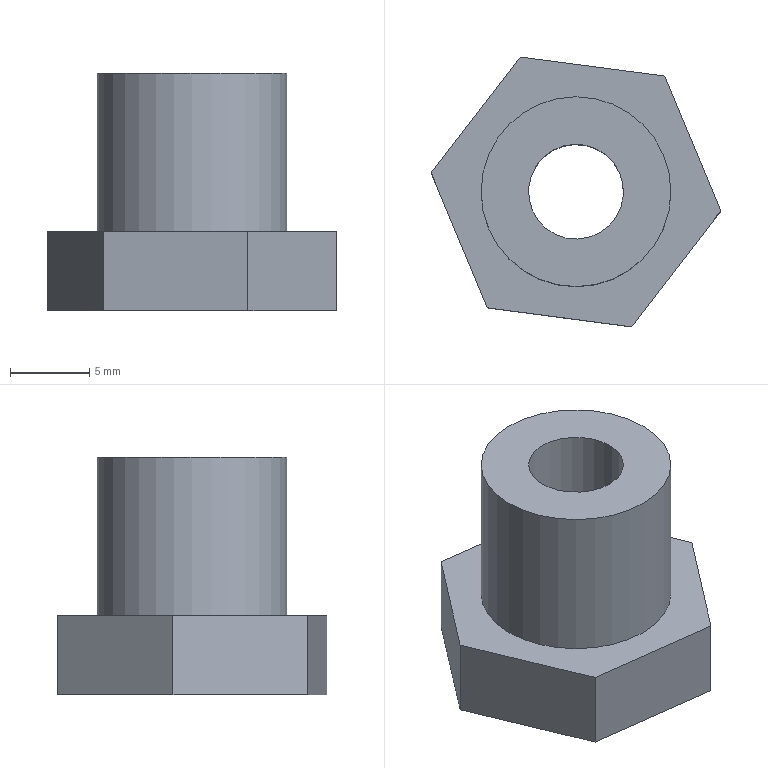Component | NX | 08__27_2 | 1 solid | 11 faces | box 18.32 x 17.07 x 15 mm | volume 1815 mm3 | plane 9 | cylinder 2 | commonest cylinder face diameters 6 x1 12 x1
STEP:
#1=CARTESIAN_POINT('',(0.,0.,0.));
#2=DIRECTION('',(0.,0.,1.));
#3=DIRECTION('',(1.,0.,0.));
#4=AXIS2_PLACEMENT_3D('',#1,#2,#3);
#5=CARTESIAN_POINT('',(110.402,102.277,172.432));
#6=VERTEX_POINT('',#5);
#7=CARTESIAN_POINT('',(106.863,110.81,172.432));
#8=VERTEX_POINT('',#7);
#9=CARTESIAN_POINT('',(110.402,102.277,172.432));
#10=DIRECTION('',(-0.383,0.9237,0.));
#11=VECTOR('',#10,1.);
#12=LINE('',#9,#11);
#13=CARTESIAN_POINT('',(110.402,102.277,167.432));
#14=DIRECTION('',(0.9237,0.383,0.));
#15=DIRECTION('',(0.383,-0.9237,0.));
#16=AXIS2_PLACEMENT_3D('',#13,#14,#15);
#17=PLANE('',#16);
#18=CARTESIAN_POINT('',(0.,-5.));
#19=DIRECTION('',(-1.,0.));
#20=VECTOR('',#19,1.);
#21=LINE('',#18,#20);
#22=(GEOMETRIC_REPRESENTATION_CONTEXT(2)PARAMETRIC_REPRESENTATION_CONTEXT()REPRESENTATION_CONTEXT('',''));
#23=DEFINITIONAL_REPRESENTATION('',(#21),#22);
#24=PCURVE('',#17,#23);
#25=CARTESIAN_POINT('',(116.022,109.608,172.432));
#26=DIRECTION('',(0.,0.,-1.));
#27=DIRECTION('',(0.9237,0.383,0.));
#28=AXIS2_PLACEMENT_3D('',#25,#26,#27);
#29=PLANE('',#28);
#30=CARTESIAN_POINT('',(-8.,4.619));
#31=DIRECTION('',(-0.,-1.));
#32=VECTOR('',#31,1.);
#33=LINE('',#30,#32);
#34=(GEOMETRIC_REPRESENTATION_CONTEXT(2)PARAMETRIC_REPRESENTATION_CONTEXT()REPRESENTATION_CONTEXT('',''));
#35=DEFINITIONAL_REPRESENTATION('',(#33),#34);
#36=PCURVE('',#29,#35);
#37=SURFACE_CURVE('',#12,(#24,#36),.PCURVE_S1.);
#38=EDGE_CURVE('',#6,#8,#37,.T.);
#39=ORIENTED_EDGE('',*,*,#38,.T.);
#40=CARTESIAN_POINT('',(106.863,110.81,167.432));
#41=VERTEX_POINT('',#40);
#42=CARTESIAN_POINT('',(106.863,110.81,167.432));
#43=DIRECTION('',(0.,0.,1.));
#44=VECTOR('',#43,1.);
#45=LINE('',#42,#44);
#46=CARTESIAN_POINT('',(-9.238,0.));
#47=DIRECTION('',(0.,-1.));
#48=VECTOR('',#47,1.);
#49=LINE('',#46,#48);
#50=(GEOMETRIC_REPRESENTATION_CONTEXT(2)PARAMETRIC_REPRESENTATION_CONTEXT()REPRESENTATION_CONTEXT('',''));
#51=DEFINITIONAL_REPRESENTATION('',(#49),#50);
#52=PCURVE('',#17,#51);
#53=CARTESIAN_POINT('',(106.863,110.81,167.432));
#54=DIRECTION('',(0.7936,-0.6084,0.));
#55=DIRECTION('',(-0.6084,-0.7936,0.));
#56=AXIS2_PLACEMENT_3D('',#53,#54,#55);
#57=PLANE('',#56);
#58=CARTESIAN_POINT('',(0.,0.));
#59=DIRECTION('',(0.,-1.));
#60=VECTOR('',#59,1.);
#61=LINE('',#58,#60);
#62=(GEOMETRIC_REPRESENTATION_CONTEXT(2)PARAMETRIC_REPRESENTATION_CONTEXT()REPRESENTATION_CONTEXT('',''));
#63=DEFINITIONAL_REPRESENTATION('',(#61),#62);
#64=PCURVE('',#57,#63);
#65=SURFACE_CURVE('',#45,(#52,#64),.PCURVE_S1.);
#66=EDGE_CURVE('',#41,#8,#65,.T.);
#67=ORIENTED_EDGE('',*,*,#66,.F.);
#68=CARTESIAN_POINT('',(110.402,102.277,167.432));
#69=VERTEX_POINT('',#68);
#70=CARTESIAN_POINT('',(110.402,102.277,167.432));
#71=DIRECTION('',(-0.383,0.9237,0.));
#72=VECTOR('',#71,1.);
#73=LINE('',#70,#72);
#74=CARTESIAN_POINT('',(0.,0.));
#75=DIRECTION('',(-1.,0.));
#76=VECTOR('',#75,1.);
#77=LINE('',#74,#76);
#78=(GEOMETRIC_REPRESENTATION_CONTEXT(2)PARAMETRIC_REPRESENTATION_CONTEXT()REPRESENTATION_CONTEXT('',''));
#79=DEFINITIONAL_REPRESENTATION('',(#77),#78);
#80=PCURVE('',#17,#79);
#81=CARTESIAN_POINT('',(116.022,109.608,167.432));
#82=DIRECTION('',(0.,0.,-1.));
#83=DIRECTION('',(0.9237,0.383,0.));
#84=AXIS2_PLACEMENT_3D('',#81,#82,#83);
#85=PLANE('',#84);
#86=CARTESIAN_POINT('',(-8.,4.619));
#87=DIRECTION('',(-0.,-1.));
#88=VECTOR('',#87,1.);
#89=LINE('',#86,#88);
#90=(GEOMETRIC_REPRESENTATION_CONTEXT(2)PARAMETRIC_REPRESENTATION_CONTEXT()REPRESENTATION_CONTEXT('',''));
#91=DEFINITIONAL_REPRESENTATION('',(#89),#90);
#92=PCURVE('',#85,#91);
#93=SURFACE_CURVE('',#73,(#80,#92),.PCURVE_S1.);
#94=EDGE_CURVE('',#69,#41,#93,.T.);
#95=ORIENTED_EDGE('',*,*,#94,.F.);
#96=CARTESIAN_POINT('',(110.402,102.277,167.432));
#97=DIRECTION('',(0.,0.,1.));
#98=VECTOR('',#97,1.);
#99=LINE('',#96,#98);
#100=CARTESIAN_POINT('',(0.,0.));
#101=DIRECTION('',(0.,-1.));
#102=VECTOR('',#101,1.);
#103=LINE('',#100,#102);
#104=(GEOMETRIC_REPRESENTATION_CONTEXT(2)PARAMETRIC_REPRESENTATION_CONTEXT()REPRESENTATION_CONTEXT('',''));
#105=DEFINITIONAL_REPRESENTATION('',(#103),#104);
#106=PCURVE('',#17,#105);
#107=CARTESIAN_POINT('',(119.561,101.075,167.432));
#108=DIRECTION('',(0.1301,0.9915,0.));
#109=DIRECTION('',(0.9915,-0.1301,0.));
#110=AXIS2_PLACEMENT_3D('',#107,#108,#109);
#111=PLANE('',#110);
#112=CARTESIAN_POINT('',(-9.238,0.));
#113=DIRECTION('',(0.,-1.));
#114=VECTOR('',#113,1.);
#115=LINE('',#112,#114);
#116=(GEOMETRIC_REPRESENTATION_CONTEXT(2)PARAMETRIC_REPRESENTATION_CONTEXT()REPRESENTATION_CONTEXT('',''));
#117=DEFINITIONAL_REPRESENTATION('',(#115),#116);
#118=PCURVE('',#111,#117);
#119=SURFACE_CURVE('',#99,(#106,#118),.PCURVE_S1.);
#120=EDGE_CURVE('',#69,#6,#119,.T.);
#121=ORIENTED_EDGE('',*,*,#120,.T.);
#122=EDGE_LOOP('',(#39,#67,#95,#121));
#123=FACE_BOUND('',#122,.T.);
#124=ADVANCED_FACE('',(#123),#17,.F.);
#125=CARTESIAN_POINT('',(112.484,118.141,172.432));
#126=VERTEX_POINT('',#125);
#127=CARTESIAN_POINT('',(106.863,110.81,172.432));
#128=DIRECTION('',(0.6084,0.7936,0.));
#129=VECTOR('',#128,1.);
#130=LINE('',#127,#129);
#131=CARTESIAN_POINT('',(0.,-5.));
#132=DIRECTION('',(-1.,0.));
#133=VECTOR('',#132,1.);
#134=LINE('',#131,#133);
#135=(GEOMETRIC_REPRESENTATION_CONTEXT(2)PARAMETRIC_REPRESENTATION_CONTEXT()REPRESENTATION_CONTEXT('',''));
#136=DEFINITIONAL_REPRESENTATION('',(#134),#135);
#137=PCURVE('',#57,#136);
#138=CARTESIAN_POINT('',(-8.,-4.619));
#139=DIRECTION('',(0.866,-0.5));
#140=VECTOR('',#139,1.);
#141=LINE('',#138,#140);
#142=(GEOMETRIC_REPRESENTATION_CONTEXT(2)PARAMETRIC_REPRESENTATION_CONTEXT()REPRESENTATION_CONTEXT('',''));
#143=DEFINITIONAL_REPRESENTATION('',(#141),#142);
#144=PCURVE('',#29,#143);
#145=SURFACE_CURVE('',#130,(#137,#144),.PCURVE_S1.);
#146=EDGE_CURVE('',#8,#126,#145,.T.);
#147=ORIENTED_EDGE('',*,*,#146,.T.);
#148=CARTESIAN_POINT('',(112.484,118.141,167.432));
#149=VERTEX_POINT('',#148);
#150=CARTESIAN_POINT('',(112.484,118.141,167.432));
#151=DIRECTION('',(0.,0.,1.));
#152=VECTOR('',#151,1.);
#153=LINE('',#150,#152);
#154=CARTESIAN_POINT('',(-9.238,0.));
#155=DIRECTION('',(0.,-1.));
#156=VECTOR('',#155,1.);
#157=LINE('',#154,#156);
#158=(GEOMETRIC_REPRESENTATION_CONTEXT(2)PARAMETRIC_REPRESENTATION_CONTEXT()REPRESENTATION_CONTEXT('',''));
#159=DEFINITIONAL_REPRESENTATION('',(#157),#158);
#160=PCURVE('',#57,#159);
#161=CARTESIAN_POINT('',(112.484,118.141,167.432));
#162=DIRECTION('',(-0.1301,-0.9915,0.));
#163=DIRECTION('',(-0.9915,0.1301,0.));
#164=AXIS2_PLACEMENT_3D('',#161,#162,#163);
#165=PLANE('',#164);
#166=CARTESIAN_POINT('',(0.,0.));
#167=DIRECTION('',(0.,-1.));
#168=VECTOR('',#167,1.);
#169=LINE('',#166,#168);
#170=(GEOMETRIC_REPRESENTATION_CONTEXT(2)PARAMETRIC_REPRESENTATION_CONTEXT()REPRESENTATION_CONTEXT('',''));
#171=DEFINITIONAL_REPRESENTATION('',(#169),#170);
#172=PCURVE('',#165,#171);
#173=SURFACE_CURVE('',#153,(#160,#172),.PCURVE_S1.);
#174=EDGE_CURVE('',#149,#126,#173,.T.);
#175=ORIENTED_EDGE('',*,*,#174,.F.);
#176=CARTESIAN_POINT('',(106.863,110.81,167.432));
#177=DIRECTION('',(0.6084,0.7936,0.));
#178=VECTOR('',#177,1.);
#179=LINE('',#176,#178);
#180=CARTESIAN_POINT('',(0.,0.));
#181=DIRECTION('',(-1.,0.));
#182=VECTOR('',#181,1.);
#183=LINE('',#180,#182);
#184=(GEOMETRIC_REPRESENTATION_CONTEXT(2)PARAMETRIC_REPRESENTATION_CONTEXT()REPRESENTATION_CONTEXT('',''));
#185=DEFINITIONAL_REPRESENTATION('',(#183),#184);
#186=PCURVE('',#57,#185);
#187=CARTESIAN_POINT('',(-8.,-4.619));
#188=DIRECTION('',(0.866,-0.5));
#189=VECTOR('',#188,1.);
#190=LINE('',#187,#189);
#191=(GEOMETRIC_REPRESENTATION_CONTEXT(2)PARAMETRIC_REPRESENTATION_CONTEXT()REPRESENTATION_CONTEXT('',''));
#192=DEFINITIONAL_REPRESENTATION('',(#190),#191);
#193=PCURVE('',#85,#192);
#194=SURFACE_CURVE('',#179,(#186,#193),.PCURVE_S1.);
#195=EDGE_CURVE('',#41,#149,#194,.T.);
#196=ORIENTED_EDGE('',*,*,#195,.F.);
#197=ORIENTED_EDGE('',*,*,#66,.T.);
#198=EDGE_LOOP('',(#147,#175,#196,#197));
#199=FACE_BOUND('',#198,.T.);
#200=ADVANCED_FACE('',(#199),#57,.F.);
#201=CARTESIAN_POINT('',(121.643,116.939,172.432));
#202=VERTEX_POINT('',#201);
#203=CARTESIAN_POINT('',(112.484,118.141,172.432));
#204=DIRECTION('',(0.9915,-0.1301,0.));
#205=VECTOR('',#204,1.);
#206=LINE('',#203,#205);
#207=CARTESIAN_POINT('',(0.,-5.));
#208=DIRECTION('',(-1.,0.));
#209=VECTOR('',#208,1.);
#210=LINE('',#207,#209);
#211=(GEOMETRIC_REPRESENTATION_CONTEXT(2)PARAMETRIC_REPRESENTATION_CONTEXT()REPRESENTATION_CONTEXT('',''));
#212=DEFINITIONAL_REPRESENTATION('',(#210),#211);
#213=PCURVE('',#165,#212);
#214=CARTESIAN_POINT('',(0.,-9.238));
#215=DIRECTION('',(0.866,0.5));
#216=VECTOR('',#215,1.);
#217=LINE('',#214,#216);
#218=(GEOMETRIC_REPRESENTATION_CONTEXT(2)PARAMETRIC_REPRESENTATION_CONTEXT()REPRESENTATION_CONTEXT('',''));
#219=DEFINITIONAL_REPRESENTATION('',(#217),#218);
#220=PCURVE('',#29,#219);
#221=SURFACE_CURVE('',#206,(#213,#220),.PCURVE_S1.);
#222=EDGE_CURVE('',#126,#202,#221,.T.);
#223=ORIENTED_EDGE('',*,*,#222,.T.);
#224=CARTESIAN_POINT('',(121.643,116.939,167.432));
#225=VERTEX_POINT('',#224);
#226=CARTESIAN_POINT('',(121.643,116.939,167.432));
#227=DIRECTION('',(0.,0.,1.));
#228=VECTOR('',#227,1.);
#229=LINE('',#226,#228);
#230=CARTESIAN_POINT('',(-9.238,0.));
#231=DIRECTION('',(0.,-1.));
#232=VECTOR('',#231,1.);
#233=LINE('',#230,#232);
#234=(GEOMETRIC_REPRESENTATION_CONTEXT(2)PARAMETRIC_REPRESENTATION_CONTEXT()REPRESENTATION_CONTEXT('',''));
#235=DEFINITIONAL_REPRESENTATION('',(#233),#234);
#236=PCURVE('',#165,#235);
#237=CARTESIAN_POINT('',(121.643,116.939,167.432));
#238=DIRECTION('',(-0.9237,-0.383,0.));
#239=DIRECTION('',(-0.383,0.9237,0.));
#240=AXIS2_PLACEMENT_3D('',#237,#238,#239);
#241=PLANE('',#240);
#242=CARTESIAN_POINT('',(0.,0.));
#243=DIRECTION('',(0.,-1.));
#244=VECTOR('',#243,1.);
#245=LINE('',#242,#244);
#246=(GEOMETRIC_REPRESENTATION_CONTEXT(2)PARAMETRIC_REPRESENTATION_CONTEXT()REPRESENTATION_CONTEXT('',''));
#247=DEFINITIONAL_REPRESENTATION('',(#245),#246);
#248=PCURVE('',#241,#247);
#249=SURFACE_CURVE('',#229,(#236,#248),.PCURVE_S1.);
#250=EDGE_CURVE('',#225,#202,#249,.T.);
#251=ORIENTED_EDGE('',*,*,#250,.F.);
#252=CARTESIAN_POINT('',(112.484,118.141,167.432));
#253=DIRECTION('',(0.9915,-0.1301,0.));
#254=VECTOR('',#253,1.);
#255=LINE('',#252,#254);
#256=CARTESIAN_POINT('',(0.,0.));
#257=DIRECTION('',(-1.,0.));
#258=VECTOR('',#257,1.);
#259=LINE('',#256,#258);
#260=(GEOMETRIC_REPRESENTATION_CONTEXT(2)PARAMETRIC_REPRESENTATION_CONTEXT()REPRESENTATION_CONTEXT('',''));
#261=DEFINITIONAL_REPRESENTATION('',(#259),#260);
#262=PCURVE('',#165,#261);
#263=CARTESIAN_POINT('',(0.,-9.238));
#264=DIRECTION('',(0.866,0.5));
#265=VECTOR('',#264,1.);
#266=LINE('',#263,#265);
#267=(GEOMETRIC_REPRESENTATION_CONTEXT(2)PARAMETRIC_REPRESENTATION_CONTEXT()REPRESENTATION_CONTEXT('',''));
#268=DEFINITIONAL_REPRESENTATION('',(#266),#267);
#269=PCURVE('',#85,#268);
#270=SURFACE_CURVE('',#255,(#262,#269),.PCURVE_S1.);
#271=EDGE_CURVE('',#149,#225,#270,.T.);
#272=ORIENTED_EDGE('',*,*,#271,.F.);
#273=ORIENTED_EDGE('',*,*,#174,.T.);
#274=EDGE_LOOP('',(#223,#251,#272,#273));
#275=FACE_BOUND('',#274,.T.);
#276=ADVANCED_FACE('',(#275),#165,.F.);
#277=CARTESIAN_POINT('',(125.181,108.406,172.432));
#278=VERTEX_POINT('',#277);
#279=CARTESIAN_POINT('',(121.643,116.939,172.432));
#280=DIRECTION('',(0.383,-0.9237,0.));
#281=VECTOR('',#280,1.);
#282=LINE('',#279,#281);
#283=CARTESIAN_POINT('',(0.,-5.));
#284=DIRECTION('',(-1.,0.));
#285=VECTOR('',#284,1.);
#286=LINE('',#283,#285);
#287=(GEOMETRIC_REPRESENTATION_CONTEXT(2)PARAMETRIC_REPRESENTATION_CONTEXT()REPRESENTATION_CONTEXT('',''));
#288=DEFINITIONAL_REPRESENTATION('',(#286),#287);
#289=PCURVE('',#241,#288);
#290=CARTESIAN_POINT('',(8.,-4.619));
#291=DIRECTION('',(0.,1.));
#292=VECTOR('',#291,1.);
#293=LINE('',#290,#292);
#294=(GEOMETRIC_REPRESENTATION_CONTEXT(2)PARAMETRIC_REPRESENTATION_CONTEXT()REPRESENTATION_CONTEXT('',''));
#295=DEFINITIONAL_REPRESENTATION('',(#293),#294);
#296=PCURVE('',#29,#295);
#297=SURFACE_CURVE('',#282,(#289,#296),.PCURVE_S1.);
#298=EDGE_CURVE('',#202,#278,#297,.T.);
#299=ORIENTED_EDGE('',*,*,#298,.T.);
#300=CARTESIAN_POINT('',(125.181,108.406,167.432));
#301=VERTEX_POINT('',#300);
#302=CARTESIAN_POINT('',(125.181,108.406,167.432));
#303=DIRECTION('',(0.,0.,1.));
#304=VECTOR('',#303,1.);
#305=LINE('',#302,#304);
#306=CARTESIAN_POINT('',(-9.238,0.));
#307=DIRECTION('',(0.,-1.));
#308=VECTOR('',#307,1.);
#309=LINE('',#306,#308);
#310=(GEOMETRIC_REPRESENTATION_CONTEXT(2)PARAMETRIC_REPRESENTATION_CONTEXT()REPRESENTATION_CONTEXT('',''));
#311=DEFINITIONAL_REPRESENTATION('',(#309),#310);
#312=PCURVE('',#241,#311);
#313=CARTESIAN_POINT('',(125.181,108.406,167.432));
#314=DIRECTION('',(-0.7936,0.6084,0.));
#315=DIRECTION('',(0.6084,0.7936,0.));
#316=AXIS2_PLACEMENT_3D('',#313,#314,#315);
#317=PLANE('',#316);
#318=CARTESIAN_POINT('',(0.,0.));
#319=DIRECTION('',(0.,-1.));
#320=VECTOR('',#319,1.);
#321=LINE('',#318,#320);
#322=(GEOMETRIC_REPRESENTATION_CONTEXT(2)PARAMETRIC_REPRESENTATION_CONTEXT()REPRESENTATION_CONTEXT('',''));
#323=DEFINITIONAL_REPRESENTATION('',(#321),#322);
#324=PCURVE('',#317,#323);
#325=SURFACE_CURVE('',#305,(#312,#324),.PCURVE_S1.);
#326=EDGE_CURVE('',#301,#278,#325,.T.);
#327=ORIENTED_EDGE('',*,*,#326,.F.);
#328=CARTESIAN_POINT('',(121.643,116.939,167.432));
#329=DIRECTION('',(0.383,-0.9237,0.));
#330=VECTOR('',#329,1.);
#331=LINE('',#328,#330);
#332=CARTESIAN_POINT('',(0.,0.));
#333=DIRECTION('',(-1.,0.));
#334=VECTOR('',#333,1.);
#335=LINE('',#332,#334);
#336=(GEOMETRIC_REPRESENTATION_CONTEXT(2)PARAMETRIC_REPRESENTATION_CONTEXT()REPRESENTATION_CONTEXT('',''));
#337=DEFINITIONAL_REPRESENTATION('',(#335),#336);
#338=PCURVE('',#241,#337);
#339=CARTESIAN_POINT('',(8.,-4.619));
#340=DIRECTION('',(0.,1.));
#341=VECTOR('',#340,1.);
#342=LINE('',#339,#341);
#343=(GEOMETRIC_REPRESENTATION_CONTEXT(2)PARAMETRIC_REPRESENTATION_CONTEXT()REPRESENTATION_CONTEXT('',''));
#344=DEFINITIONAL_REPRESENTATION('',(#342),#343);
#345=PCURVE('',#85,#344);
#346=SURFACE_CURVE('',#331,(#338,#345),.PCURVE_S1.);
#347=EDGE_CURVE('',#225,#301,#346,.T.);
#348=ORIENTED_EDGE('',*,*,#347,.F.);
#349=ORIENTED_EDGE('',*,*,#250,.T.);
#350=EDGE_LOOP('',(#299,#327,#348,#349));
#351=FACE_BOUND('',#350,.T.);
#352=ADVANCED_FACE('',(#351),#241,.F.);
#353=CARTESIAN_POINT('',(119.561,101.075,172.432));
#354=VERTEX_POINT('',#353);
#355=CARTESIAN_POINT('',(125.181,108.406,172.432));
#356=DIRECTION('',(-0.6084,-0.7936,0.));
#357=VECTOR('',#356,1.);
#358=LINE('',#355,#357);
#359=CARTESIAN_POINT('',(0.,-5.));
#360=DIRECTION('',(-1.,0.));
#361=VECTOR('',#360,1.);
#362=LINE('',#359,#361);
#363=(GEOMETRIC_REPRESENTATION_CONTEXT(2)PARAMETRIC_REPRESENTATION_CONTEXT()REPRESENTATION_CONTEXT('',''));
#364=DEFINITIONAL_REPRESENTATION('',(#362),#363);
#365=PCURVE('',#317,#364);
#366=CARTESIAN_POINT('',(8.,4.619));
#367=DIRECTION('',(-0.866,0.5));
#368=VECTOR('',#367,1.);
#369=LINE('',#366,#368);
#370=(GEOMETRIC_REPRESENTATION_CONTEXT(2)PARAMETRIC_REPRESENTATION_CONTEXT()REPRESENTATION_CONTEXT('',''));
#371=DEFINITIONAL_REPRESENTATION('',(#369),#370);
#372=PCURVE('',#29,#371);
#373=SURFACE_CURVE('',#358,(#365,#372),.PCURVE_S1.);
#374=EDGE_CURVE('',#278,#354,#373,.T.);
#375=ORIENTED_EDGE('',*,*,#374,.T.);
#376=CARTESIAN_POINT('',(119.561,101.075,167.432));
#377=VERTEX_POINT('',#376);
#378=CARTESIAN_POINT('',(119.561,101.075,167.432));
#379=DIRECTION('',(0.,0.,1.));
#380=VECTOR('',#379,1.);
#381=LINE('',#378,#380);
#382=CARTESIAN_POINT('',(-9.238,0.));
#383=DIRECTION('',(0.,-1.));
#384=VECTOR('',#383,1.);
#385=LINE('',#382,#384);
#386=(GEOMETRIC_REPRESENTATION_CONTEXT(2)PARAMETRIC_REPRESENTATION_CONTEXT()REPRESENTATION_CONTEXT('',''));
#387=DEFINITIONAL_REPRESENTATION('',(#385),#386);
#388=PCURVE('',#317,#387);
#389=CARTESIAN_POINT('',(0.,0.));
#390=DIRECTION('',(0.,-1.));
#391=VECTOR('',#390,1.);
#392=LINE('',#389,#391);
#393=(GEOMETRIC_REPRESENTATION_CONTEXT(2)PARAMETRIC_REPRESENTATION_CONTEXT()REPRESENTATION_CONTEXT('',''));
#394=DEFINITIONAL_REPRESENTATION('',(#392),#393);
#395=PCURVE('',#111,#394);
#396=SURFACE_CURVE('',#381,(#388,#395),.PCURVE_S1.);
#397=EDGE_CURVE('',#377,#354,#396,.T.);
#398=ORIENTED_EDGE('',*,*,#397,.F.);
#399=CARTESIAN_POINT('',(125.181,108.406,167.432));
#400=DIRECTION('',(-0.6084,-0.7936,0.));
#401=VECTOR('',#400,1.);
#402=LINE('',#399,#401);
#403=CARTESIAN_POINT('',(0.,0.));
#404=DIRECTION('',(-1.,0.));
#405=VECTOR('',#404,1.);
#406=LINE('',#403,#405);
#407=(GEOMETRIC_REPRESENTATION_CONTEXT(2)PARAMETRIC_REPRESENTATION_CONTEXT()REPRESENTATION_CONTEXT('',''));
#408=DEFINITIONAL_REPRESENTATION('',(#406),#407);
#409=PCURVE('',#317,#408);
#410=CARTESIAN_POINT('',(8.,4.619));
#411=DIRECTION('',(-0.866,0.5));
#412=VECTOR('',#411,1.);
#413=LINE('',#410,#412);
#414=(GEOMETRIC_REPRESENTATION_CONTEXT(2)PARAMETRIC_REPRESENTATION_CONTEXT()REPRESENTATION_CONTEXT('',''));
#415=DEFINITIONAL_REPRESENTATION('',(#413),#414);
#416=PCURVE('',#85,#415);
#417=SURFACE_CURVE('',#402,(#409,#416),.PCURVE_S1.);
#418=EDGE_CURVE('',#301,#377,#417,.T.);
#419=ORIENTED_EDGE('',*,*,#418,.F.);
#420=ORIENTED_EDGE('',*,*,#326,.T.);
#421=EDGE_LOOP('',(#375,#398,#419,#420));
#422=FACE_BOUND('',#421,.T.);
#423=ADVANCED_FACE('',(#422),#317,.F.);
#424=CARTESIAN_POINT('',(119.561,101.075,172.432));
#425=DIRECTION('',(-0.9915,0.1301,0.));
#426=VECTOR('',#425,1.);
#427=LINE('',#424,#426);
#428=CARTESIAN_POINT('',(0.,-5.));
#429=DIRECTION('',(-1.,0.));
#430=VECTOR('',#429,1.);
#431=LINE('',#428,#430);
#432=(GEOMETRIC_REPRESENTATION_CONTEXT(2)PARAMETRIC_REPRESENTATION_CONTEXT()REPRESENTATION_CONTEXT('',''));
#433=DEFINITIONAL_REPRESENTATION('',(#431),#432);
#434=PCURVE('',#111,#433);
#435=CARTESIAN_POINT('',(-0.,9.238));
#436=DIRECTION('',(-0.866,-0.5));
#437=VECTOR('',#436,1.);
#438=LINE('',#435,#437);
#439=(GEOMETRIC_REPRESENTATION_CONTEXT(2)PARAMETRIC_REPRESENTATION_CONTEXT()REPRESENTATION_CONTEXT('',''));
#440=DEFINITIONAL_REPRESENTATION('',(#438),#439);
#441=PCURVE('',#29,#440);
#442=SURFACE_CURVE('',#427,(#434,#441),.PCURVE_S1.);
#443=EDGE_CURVE('',#354,#6,#442,.T.);
#444=ORIENTED_EDGE('',*,*,#443,.T.);
#445=ORIENTED_EDGE('',*,*,#120,.F.);
#446=CARTESIAN_POINT('',(119.561,101.075,167.432));
#447=DIRECTION('',(-0.9915,0.1301,0.));
#448=VECTOR('',#447,1.);
#449=LINE('',#446,#448);
#450=CARTESIAN_POINT('',(0.,0.));
#451=DIRECTION('',(-1.,0.));
#452=VECTOR('',#451,1.);
#453=LINE('',#450,#452);
#454=(GEOMETRIC_REPRESENTATION_CONTEXT(2)PARAMETRIC_REPRESENTATION_CONTEXT()REPRESENTATION_CONTEXT('',''));
#455=DEFINITIONAL_REPRESENTATION('',(#453),#454);
#456=PCURVE('',#111,#455);
#457=CARTESIAN_POINT('',(-0.,9.238));
#458=DIRECTION('',(-0.866,-0.5));
#459=VECTOR('',#458,1.);
#460=LINE('',#457,#459);
#461=(GEOMETRIC_REPRESENTATION_CONTEXT(2)PARAMETRIC_REPRESENTATION_CONTEXT()REPRESENTATION_CONTEXT('',''));
#462=DEFINITIONAL_REPRESENTATION('',(#460),#461);
#463=PCURVE('',#85,#462);
#464=SURFACE_CURVE('',#449,(#456,#463),.PCURVE_S1.);
#465=EDGE_CURVE('',#377,#69,#464,.T.);
#466=ORIENTED_EDGE('',*,*,#465,.F.);
#467=ORIENTED_EDGE('',*,*,#397,.T.);
#468=EDGE_LOOP('',(#444,#445,#466,#467));
#469=FACE_BOUND('',#468,.T.);
#470=ADVANCED_FACE('',(#469),#111,.F.);
#471=CARTESIAN_POINT('',(118.793,110.757,167.432));
#472=VERTEX_POINT('',#471);
#473=CARTESIAN_POINT('',(116.022,109.608,167.432));
#474=DIRECTION('',(0.,0.,-1.));
#475=DIRECTION('',(0.9237,0.383,0.));
#476=AXIS2_PLACEMENT_3D('',#473,#474,#475);
#477=CIRCLE('',#476,3.);
#478=CARTESIAN_POINT('',(116.022,109.608,167.432));
#479=DIRECTION('',(0.,0.,1.));
#480=DIRECTION('',(-0.9237,-0.383,0.));
#481=AXIS2_PLACEMENT_3D('',#478,#479,#480);
#482=CYLINDRICAL_SURFACE('',#481,3.);
#483=CARTESIAN_POINT('',(9.425,0.));
#484=DIRECTION('',(-1.,0.));
#485=VECTOR('',#484,1.);
#486=LINE('',#483,#485);
#487=(GEOMETRIC_REPRESENTATION_CONTEXT(2)PARAMETRIC_REPRESENTATION_CONTEXT()REPRESENTATION_CONTEXT('',''));
#488=DEFINITIONAL_REPRESENTATION('',(#486),#487);
#489=PCURVE('',#482,#488);
#490=CARTESIAN_POINT('',(0.,0.));
#491=DIRECTION('',(1.,-0.));
#492=AXIS2_PLACEMENT_2D('',#490,#491);
#493=CIRCLE('',#492,3.);
#494=(GEOMETRIC_REPRESENTATION_CONTEXT(2)PARAMETRIC_REPRESENTATION_CONTEXT()REPRESENTATION_CONTEXT('',''));
#495=DEFINITIONAL_REPRESENTATION('',(#493),#494);
#496=PCURVE('',#85,#495);
#497=SURFACE_CURVE('',#477,(#489,#496),.PCURVE_S1.);
#498=EDGE_CURVE('',#472,#472,#497,.T.);
#499=ORIENTED_EDGE('',*,*,#498,.F.);
#500=CARTESIAN_POINT('',(118.793,110.757,182.432));
#501=VERTEX_POINT('',#500);
#502=CARTESIAN_POINT('',(118.793,110.757,167.432));
#503=CARTESIAN_POINT('',(118.793,110.757,182.432));
#504=B_SPLINE_CURVE_WITH_KNOTS('',1,(#502,#503),.UNSPECIFIED.,.F.,.F.,(2,2),(0.,15.),.PIECEWISE_BEZIER_KNOTS.);
#505=CARTESIAN_POINT('',(9.425,0.));
#506=DIRECTION('',(0.,1.));
#507=VECTOR('',#506,1.);
#508=LINE('',#505,#507);
#509=(GEOMETRIC_REPRESENTATION_CONTEXT(2)PARAMETRIC_REPRESENTATION_CONTEXT()REPRESENTATION_CONTEXT('',''));
#510=DEFINITIONAL_REPRESENTATION('',(#508),#509);
#511=PCURVE('',#482,#510);
#512=CARTESIAN_POINT('',(3.142,0.));
#513=DIRECTION('',(0.,1.));
#514=VECTOR('',#513,1.);
#515=LINE('',#512,#514);
#516=(GEOMETRIC_REPRESENTATION_CONTEXT(2)PARAMETRIC_REPRESENTATION_CONTEXT()REPRESENTATION_CONTEXT('',''));
#517=DEFINITIONAL_REPRESENTATION('',(#515),#516);
#518=PCURVE('',#482,#517);
#519=SEAM_CURVE('',#504,(#511,#518),.PCURVE_S1.);
#520=EDGE_CURVE('',#472,#501,#519,.T.);
#521=ORIENTED_EDGE('',*,*,#520,.T.);
#522=CARTESIAN_POINT('',(116.022,109.608,182.432));
#523=DIRECTION('',(0.,0.,-1.));
#524=DIRECTION('',(0.9237,0.383,0.));
#525=AXIS2_PLACEMENT_3D('',#522,#523,#524);
#526=CIRCLE('',#525,3.);
#527=CARTESIAN_POINT('',(9.425,15.));
#528=DIRECTION('',(-1.,0.));
#529=VECTOR('',#528,1.);
#530=LINE('',#527,#529);
#531=(GEOMETRIC_REPRESENTATION_CONTEXT(2)PARAMETRIC_REPRESENTATION_CONTEXT()REPRESENTATION_CONTEXT('',''));
#532=DEFINITIONAL_REPRESENTATION('',(#530),#531);
#533=PCURVE('',#482,#532);
#534=CARTESIAN_POINT('',(116.022,109.608,182.432));
#535=DIRECTION('',(0.,0.,-1.));
#536=DIRECTION('',(0.9237,0.383,0.));
#537=AXIS2_PLACEMENT_3D('',#534,#535,#536);
#538=PLANE('',#537);
#539=CARTESIAN_POINT('',(0.,0.));
#540=DIRECTION('',(1.,-0.));
#541=AXIS2_PLACEMENT_2D('',#539,#540);
#542=CIRCLE('',#541,3.);
#543=(GEOMETRIC_REPRESENTATION_CONTEXT(2)PARAMETRIC_REPRESENTATION_CONTEXT()REPRESENTATION_CONTEXT('',''));
#544=DEFINITIONAL_REPRESENTATION('',(#542),#543);
#545=PCURVE('',#538,#544);
#546=SURFACE_CURVE('',#526,(#533,#545),.PCURVE_S1.);
#547=EDGE_CURVE('',#501,#501,#546,.T.);
#548=ORIENTED_EDGE('',*,*,#547,.T.);
#549=ORIENTED_EDGE('',*,*,#520,.F.);
#550=EDGE_LOOP('',(#499,#521,#548,#549));
#551=FACE_BOUND('',#550,.F.);
#552=ADVANCED_FACE('',(#551),#482,.F.);
#553=ORIENTED_EDGE('',*,*,#94,.T.);
#554=ORIENTED_EDGE('',*,*,#195,.T.);
#555=ORIENTED_EDGE('',*,*,#271,.T.);
#556=ORIENTED_EDGE('',*,*,#347,.T.);
#557=ORIENTED_EDGE('',*,*,#418,.T.);
#558=ORIENTED_EDGE('',*,*,#465,.T.);
#559=EDGE_LOOP('',(#553,#554,#555,#556,#557,#558));
#560=FACE_BOUND('',#559,.T.);
#561=ORIENTED_EDGE('',*,*,#498,.F.);
#562=EDGE_LOOP('',(#561));
#563=FACE_BOUND('',#562,.T.);
#564=ADVANCED_FACE('',(#560,#563),#85,.T.);
#565=CARTESIAN_POINT('',(121.565,111.906,172.432));
#566=VERTEX_POINT('',#565);
#567=CARTESIAN_POINT('',(116.022,109.608,172.432));
#568=DIRECTION('',(0.,0.,-1.));
#569=DIRECTION('',(0.9237,0.383,0.));
#570=AXIS2_PLACEMENT_3D('',#567,#568,#569);
#571=CIRCLE('',#570,6.);
#572=CARTESIAN_POINT('',(0.,0.));
#573=DIRECTION('',(1.,0.));
#574=AXIS2_PLACEMENT_2D('',#572,#573);
#575=CIRCLE('',#574,6.);
#576=(GEOMETRIC_REPRESENTATION_CONTEXT(2)PARAMETRIC_REPRESENTATION_CONTEXT()REPRESENTATION_CONTEXT('',''));
#577=DEFINITIONAL_REPRESENTATION('',(#575),#576);
#578=PCURVE('',#29,#577);
#579=CARTESIAN_POINT('',(116.022,109.608,182.432));
#580=DIRECTION('',(0.,0.,-1.));
#581=DIRECTION('',(0.9237,0.383,0.));
#582=AXIS2_PLACEMENT_3D('',#579,#580,#581);
#583=CYLINDRICAL_SURFACE('',#582,6.);
#584=CARTESIAN_POINT('',(0.,10.));
#585=DIRECTION('',(1.,0.));
#586=VECTOR('',#585,1.);
#587=LINE('',#584,#586);
#588=(GEOMETRIC_REPRESENTATION_CONTEXT(2)PARAMETRIC_REPRESENTATION_CONTEXT()REPRESENTATION_CONTEXT('',''));
#589=DEFINITIONAL_REPRESENTATION('',(#587),#588);
#590=PCURVE('',#583,#589);
#591=SURFACE_CURVE('',#571,(#578,#590),.PCURVE_S1.);
#592=EDGE_CURVE('',#566,#566,#591,.T.);
#593=ORIENTED_EDGE('',*,*,#592,.T.);
#594=EDGE_LOOP('',(#593));
#595=FACE_BOUND('',#594,.T.);
#596=ORIENTED_EDGE('',*,*,#38,.F.);
#597=ORIENTED_EDGE('',*,*,#443,.F.);
#598=ORIENTED_EDGE('',*,*,#374,.F.);
#599=ORIENTED_EDGE('',*,*,#298,.F.);
#600=ORIENTED_EDGE('',*,*,#222,.F.);
#601=ORIENTED_EDGE('',*,*,#146,.F.);
#602=EDGE_LOOP('',(#596,#597,#598,#599,#600,#601));
#603=FACE_BOUND('',#602,.T.);
#604=ADVANCED_FACE('',(#595,#603),#29,.F.);
#605=CARTESIAN_POINT('',(121.565,111.906,182.432));
#606=VERTEX_POINT('',#605);
#607=CARTESIAN_POINT('',(116.022,109.608,182.432));
#608=DIRECTION('',(0.,0.,-1.));
#609=DIRECTION('',(0.9237,0.383,0.));
#610=AXIS2_PLACEMENT_3D('',#607,#608,#609);
#611=CIRCLE('',#610,6.);
#612=CARTESIAN_POINT('',(0.,0.));
#613=DIRECTION('',(1.,0.));
#614=VECTOR('',#613,1.);
#615=LINE('',#612,#614);
#616=(GEOMETRIC_REPRESENTATION_CONTEXT(2)PARAMETRIC_REPRESENTATION_CONTEXT()REPRESENTATION_CONTEXT('',''));
#617=DEFINITIONAL_REPRESENTATION('',(#615),#616);
#618=PCURVE('',#583,#617);
#619=CARTESIAN_POINT('',(0.,0.));
#620=DIRECTION('',(1.,0.));
#621=AXIS2_PLACEMENT_2D('',#619,#620);
#622=CIRCLE('',#621,6.);
#623=(GEOMETRIC_REPRESENTATION_CONTEXT(2)PARAMETRIC_REPRESENTATION_CONTEXT()REPRESENTATION_CONTEXT('',''));
#624=DEFINITIONAL_REPRESENTATION('',(#622),#623);
#625=PCURVE('',#538,#624);
#626=SURFACE_CURVE('',#611,(#618,#625),.PCURVE_S1.);
#627=EDGE_CURVE('',#606,#606,#626,.T.);
#628=ORIENTED_EDGE('',*,*,#627,.T.);
#629=CARTESIAN_POINT('',(121.565,111.906,182.432));
#630=CARTESIAN_POINT('',(121.565,111.906,172.432));
#631=B_SPLINE_CURVE_WITH_KNOTS('',1,(#629,#630),.UNSPECIFIED.,.F.,.F.,(2,2),(0.,10.),.PIECEWISE_BEZIER_KNOTS.);
#632=CARTESIAN_POINT('',(6.283,0.));
#633=DIRECTION('',(0.,1.));
#634=VECTOR('',#633,1.);
#635=LINE('',#632,#634);
#636=(GEOMETRIC_REPRESENTATION_CONTEXT(2)PARAMETRIC_REPRESENTATION_CONTEXT()REPRESENTATION_CONTEXT('',''));
#637=DEFINITIONAL_REPRESENTATION('',(#635),#636);
#638=PCURVE('',#583,#637);
#639=CARTESIAN_POINT('',(0.,0.));
#640=DIRECTION('',(0.,1.));
#641=VECTOR('',#640,1.);
#642=LINE('',#639,#641);
#643=(GEOMETRIC_REPRESENTATION_CONTEXT(2)PARAMETRIC_REPRESENTATION_CONTEXT()REPRESENTATION_CONTEXT('',''));
#644=DEFINITIONAL_REPRESENTATION('',(#642),#643);
#645=PCURVE('',#583,#644);
#646=SEAM_CURVE('',#631,(#638,#645),.PCURVE_S1.);
#647=EDGE_CURVE('',#606,#566,#646,.T.);
#648=ORIENTED_EDGE('',*,*,#647,.T.);
#649=ORIENTED_EDGE('',*,*,#592,.F.);
#650=ORIENTED_EDGE('',*,*,#647,.F.);
#651=EDGE_LOOP('',(#628,#648,#649,#650));
#652=FACE_BOUND('',#651,.T.);
#653=ADVANCED_FACE('',(#652),#583,.T.);
#654=ORIENTED_EDGE('',*,*,#627,.F.);
#655=EDGE_LOOP('',(#654));
#656=FACE_BOUND('',#655,.T.);
#657=ORIENTED_EDGE('',*,*,#547,.T.);
#658=EDGE_LOOP('',(#657));
#659=FACE_BOUND('',#658,.T.);
#660=ADVANCED_FACE('',(#656,#659),#538,.F.);
#661=CLOSED_SHELL('',(#124,#200,#276,#352,#423,#470,#552,#564,#604,#653,#660));
#662=MANIFOLD_SOLID_BREP('',#661);
#663=(LENGTH_UNIT()NAMED_UNIT(*)SI_UNIT(.MILLI.,.METRE.));
#664=UNCERTAINTY_MEASURE_WITH_UNIT(LENGTH_MEASURE(0.000002),#663,'','');
#665=(NAMED_UNIT(*)PLANE_ANGLE_UNIT()SI_UNIT($,.RADIAN.));
#666=(NAMED_UNIT(*)SI_UNIT($,.STERADIAN.)SOLID_ANGLE_UNIT());
#667=(GEOMETRIC_REPRESENTATION_CONTEXT(3)GLOBAL_UNCERTAINTY_ASSIGNED_CONTEXT((#664))GLOBAL_UNIT_ASSIGNED_CONTEXT((#663,#665,#666))REPRESENTATION_CONTEXT('',''));
#668=ADVANCED_BREP_SHAPE_REPRESENTATION('',(#4,#662),#667);